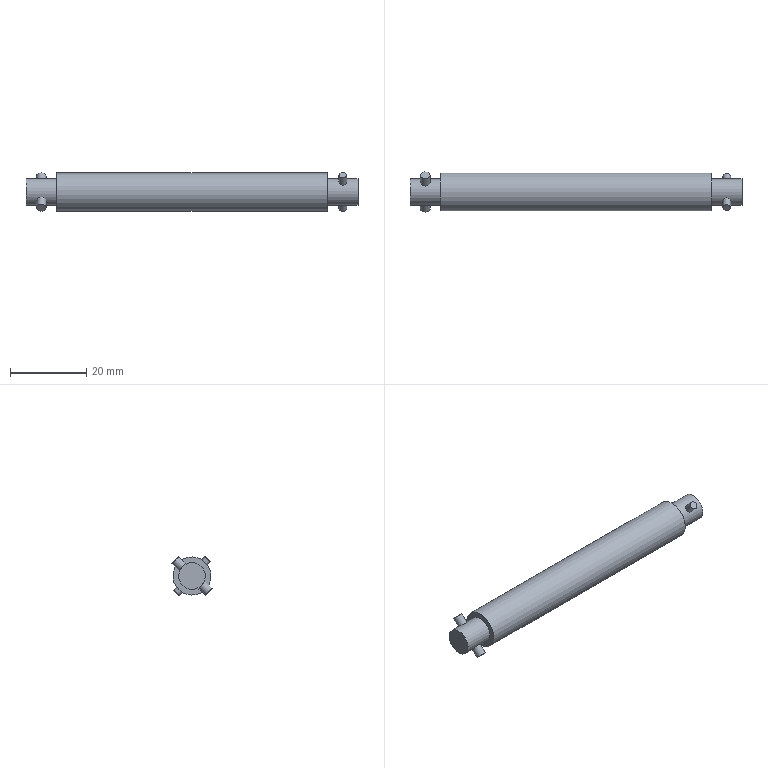Component | NX | 15C__27 | 1 solid | 15 faces | volume 6233 mm3 | plane 8 | cylinder 7 | commonest cylinder face diameters 7 x2 2.5 x2 2 x2 10 x1